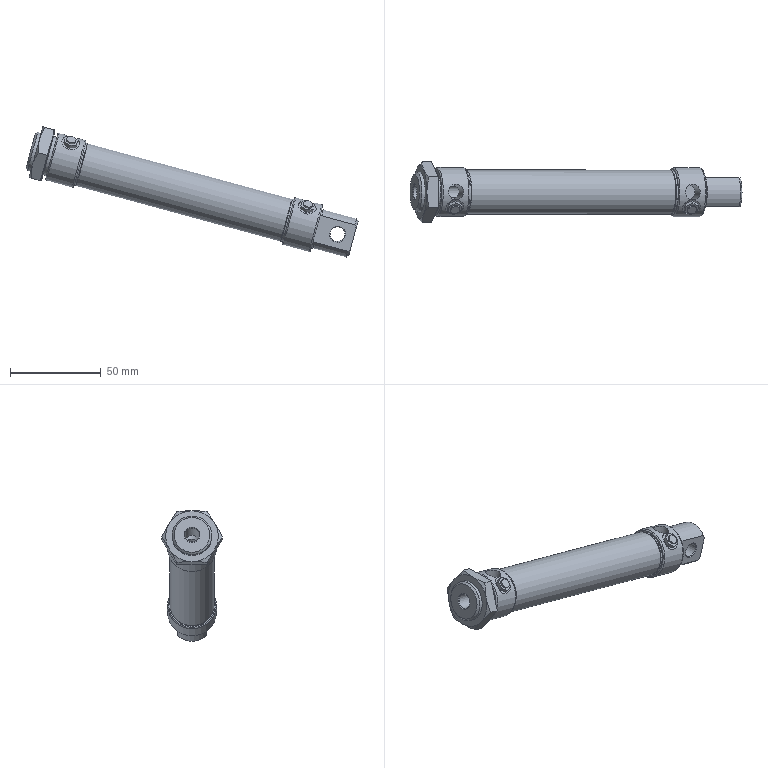Component | NX | HMAC_GT | 2 solids | 85 faces | volume 79189 mm3 | plane 43 | cylinder 26 | cone 12 | torus 4 | commonest cylinder face diameters 22 x7 10.2 x4 8.566 x3 24.3 x3 27 x2 23.7 x2 8 x2 5.1 x2